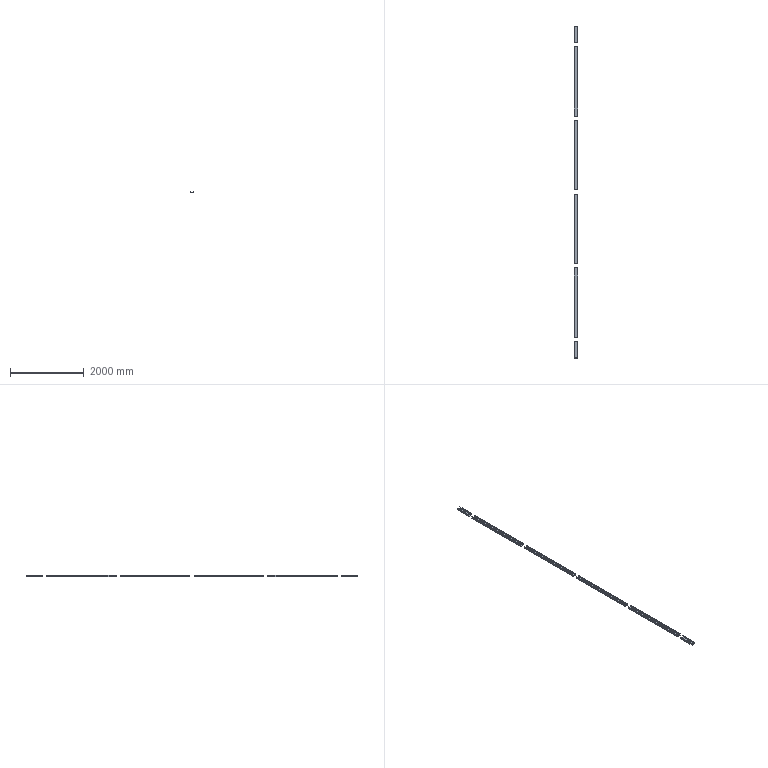Component | NX | CHUNSHUIJINCAO_CAOGANG1 | 6 solids | 60 faces | volume 10562119 mm3 | plane 60